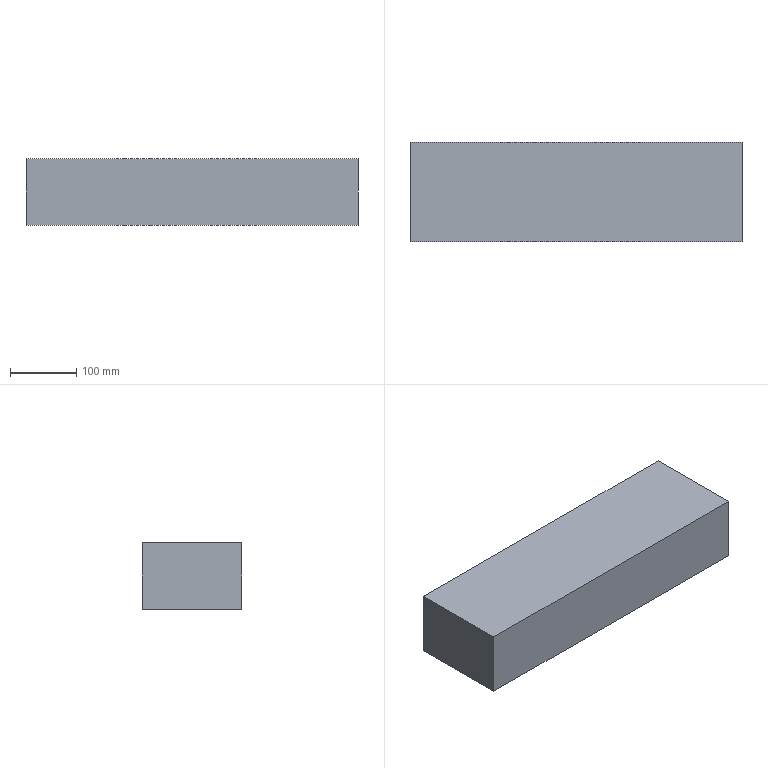Component | SolidWorks | ShadowlessLamp-B-1 | 1 solid | 6 faces | box 500 x 150 x 100 mm | volume 7500000 mm3 | plane 6
build123d program:
from build123d import *

# Parameters (mm, degrees)
SKETCH1_W           = 500
SKETCH1_H           = 100
BOSS_EXTRUDE1_DEPTH = 150


with BuildPart() as part:
    # Sketch1 → Boss-Extrude1 (new body)
    with BuildSketch(Plane.XY):
        Rectangle(SKETCH1_W, SKETCH1_H)
    extrude(amount=BOSS_EXTRUDE1_DEPTH)


solid = part.part

# Placed as in the assembly
solid = solid.moved(Location((-443.006, -571.913, -2307.928), (90, 0, 0)))
STEP:
#1=COLOUR_RGB('',0.7922,0.8196,0.9333);
#2=FILL_AREA_STYLE_COLOUR('',#1);
#3=FILL_AREA_STYLE('',(#2));
#4=SURFACE_STYLE_FILL_AREA(#3);
#5=SURFACE_SIDE_STYLE('',(#4));
#6=SURFACE_STYLE_USAGE(.BOTH.,#5);
#7=PRESENTATION_STYLE_ASSIGNMENT((#6));
#8=CARTESIAN_POINT('',(-7.599,-22.516,-92.832));
#9=VERTEX_POINT('',#8);
#10=CARTESIAN_POINT('',(-7.599,-22.516,-88.895));
#11=VERTEX_POINT('',#10);
#12=CARTESIAN_POINT('',(-7.599,-22.516,-88.895));
#13=DIRECTION('',(0.,-0.,1.));
#14=VECTOR('',#13,39.37);
#15=LINE('',#12,#14);
#16=EDGE_CURVE('',#9,#11,#15,.T.);
#17=ORIENTED_EDGE('',*,*,#16,.T.);
#18=CARTESIAN_POINT('',(-7.599,-28.422,-88.895));
#19=VERTEX_POINT('',#18);
#20=CARTESIAN_POINT('',(-7.599,-28.422,-88.895));
#21=DIRECTION('',(0.,1.,0.));
#22=VECTOR('',#21,39.37);
#23=LINE('',#20,#22);
#24=EDGE_CURVE('',#19,#11,#23,.T.);
#25=ORIENTED_EDGE('',*,*,#24,.F.);
#26=CARTESIAN_POINT('',(-7.599,-28.422,-92.832));
#27=VERTEX_POINT('',#26);
#28=CARTESIAN_POINT('',(-7.599,-28.422,-88.895));
#29=DIRECTION('',(0.,-0.,1.));
#30=VECTOR('',#29,39.37);
#31=LINE('',#28,#30);
#32=EDGE_CURVE('',#27,#19,#31,.T.);
#33=ORIENTED_EDGE('',*,*,#32,.F.);
#34=CARTESIAN_POINT('',(-7.599,-28.422,-92.832));
#35=DIRECTION('',(0.,1.,0.));
#36=VECTOR('',#35,39.37);
#37=LINE('',#34,#36);
#38=EDGE_CURVE('',#27,#9,#37,.T.);
#39=ORIENTED_EDGE('',*,*,#38,.T.);
#40=EDGE_LOOP('',(#17,#25,#33,#39));
#41=FACE_OUTER_BOUND('',#40,.T.);
#42=CARTESIAN_POINT('',(-7.599,-28.422,-88.895));
#43=DIRECTION('',(-1.,0.,0.));
#44=DIRECTION('',(-0.,-1.,-0.));
#45=AXIS2_PLACEMENT_3D('',#42,#43,#44);
#46=PLANE('',#45);
#47=ADVANCED_FACE('',(#41),#46,.F.);
#48=CARTESIAN_POINT('',(-27.284,-22.516,-88.895));
#49=VERTEX_POINT('',#48);
#50=CARTESIAN_POINT('',(-27.284,-22.516,-88.895));
#51=DIRECTION('',(-1.,0.,0.));
#52=VECTOR('',#51,39.37);
#53=LINE('',#50,#52);
#54=EDGE_CURVE('',#11,#49,#53,.T.);
#55=ORIENTED_EDGE('',*,*,#54,.T.);
#56=CARTESIAN_POINT('',(-27.284,-28.422,-88.895));
#57=VERTEX_POINT('',#56);
#58=CARTESIAN_POINT('',(-27.284,-28.422,-88.895));
#59=DIRECTION('',(0.,1.,0.));
#60=VECTOR('',#59,39.37);
#61=LINE('',#58,#60);
#62=EDGE_CURVE('',#57,#49,#61,.T.);
#63=ORIENTED_EDGE('',*,*,#62,.F.);
#64=CARTESIAN_POINT('',(-27.284,-28.422,-88.895));
#65=DIRECTION('',(-1.,0.,0.));
#66=VECTOR('',#65,39.37);
#67=LINE('',#64,#66);
#68=EDGE_CURVE('',#19,#57,#67,.T.);
#69=ORIENTED_EDGE('',*,*,#68,.F.);
#70=ORIENTED_EDGE('',*,*,#24,.T.);
#71=EDGE_LOOP('',(#55,#63,#69,#70));
#72=FACE_OUTER_BOUND('',#71,.T.);
#73=CARTESIAN_POINT('',(-27.284,-28.422,-88.895));
#74=DIRECTION('',(-0.,0.,-1.));
#75=DIRECTION('',(0.,1.,0.));
#76=AXIS2_PLACEMENT_3D('',#73,#74,#75);
#77=PLANE('',#76);
#78=ADVANCED_FACE('',(#72),#77,.F.);
#79=CARTESIAN_POINT('',(-27.284,-22.516,-92.832));
#80=VERTEX_POINT('',#79);
#81=CARTESIAN_POINT('',(-27.284,-22.516,-88.895));
#82=DIRECTION('',(-0.,0.,-1.));
#83=VECTOR('',#82,39.37);
#84=LINE('',#81,#83);
#85=EDGE_CURVE('',#49,#80,#84,.T.);
#86=ORIENTED_EDGE('',*,*,#85,.T.);
#87=CARTESIAN_POINT('',(-27.284,-28.422,-92.832));
#88=VERTEX_POINT('',#87);
#89=CARTESIAN_POINT('',(-27.284,-28.422,-92.832));
#90=DIRECTION('',(0.,1.,0.));
#91=VECTOR('',#90,39.37);
#92=LINE('',#89,#91);
#93=EDGE_CURVE('',#88,#80,#92,.T.);
#94=ORIENTED_EDGE('',*,*,#93,.F.);
#95=CARTESIAN_POINT('',(-27.284,-28.422,-88.895));
#96=DIRECTION('',(-0.,0.,-1.));
#97=VECTOR('',#96,39.37);
#98=LINE('',#95,#97);
#99=EDGE_CURVE('',#57,#88,#98,.T.);
#100=ORIENTED_EDGE('',*,*,#99,.F.);
#101=ORIENTED_EDGE('',*,*,#62,.T.);
#102=EDGE_LOOP('',(#86,#94,#100,#101));
#103=FACE_OUTER_BOUND('',#102,.T.);
#104=CARTESIAN_POINT('',(-27.284,-28.422,-88.895));
#105=DIRECTION('',(1.,-0.,-0.));
#106=DIRECTION('',(0.,1.,0.));
#107=AXIS2_PLACEMENT_3D('',#104,#105,#106);
#108=PLANE('',#107);
#109=ADVANCED_FACE('',(#103),#108,.F.);
#110=CARTESIAN_POINT('',(-27.284,-22.516,-92.832));
#111=DIRECTION('',(1.,-0.,-0.));
#112=VECTOR('',#111,39.37);
#113=LINE('',#110,#112);
#114=EDGE_CURVE('',#80,#9,#113,.T.);
#115=ORIENTED_EDGE('',*,*,#114,.T.);
#116=ORIENTED_EDGE('',*,*,#38,.F.);
#117=CARTESIAN_POINT('',(-27.284,-28.422,-92.832));
#118=DIRECTION('',(1.,-0.,-0.));
#119=VECTOR('',#118,39.37);
#120=LINE('',#117,#119);
#121=EDGE_CURVE('',#88,#27,#120,.T.);
#122=ORIENTED_EDGE('',*,*,#121,.F.);
#123=ORIENTED_EDGE('',*,*,#93,.T.);
#124=EDGE_LOOP('',(#115,#116,#122,#123));
#125=FACE_OUTER_BOUND('',#124,.T.);
#126=CARTESIAN_POINT('',(-27.284,-28.422,-92.832));
#127=DIRECTION('',(0.,-0.,1.));
#128=DIRECTION('',(-0.,-1.,-0.));
#129=AXIS2_PLACEMENT_3D('',#126,#127,#128);
#130=PLANE('',#129);
#131=ADVANCED_FACE('',(#125),#130,.F.);
#132=ORIENTED_EDGE('',*,*,#32,.T.);
#133=ORIENTED_EDGE('',*,*,#68,.T.);
#134=ORIENTED_EDGE('',*,*,#99,.T.);
#135=ORIENTED_EDGE('',*,*,#121,.T.);
#136=EDGE_LOOP('',(#132,#133,#134,#135));
#137=FACE_OUTER_BOUND('',#136,.T.);
#138=CARTESIAN_POINT('',(-17.441,-28.422,-90.863));
#139=DIRECTION('',(-0.,-1.,-0.));
#140=DIRECTION('',(1.,-0.,-0.));
#141=AXIS2_PLACEMENT_3D('',#138,#139,#140);
#142=PLANE('',#141);
#143=ADVANCED_FACE('',(#137),#142,.T.);
#144=ORIENTED_EDGE('',*,*,#16,.F.);
#145=ORIENTED_EDGE('',*,*,#114,.F.);
#146=ORIENTED_EDGE('',*,*,#85,.F.);
#147=ORIENTED_EDGE('',*,*,#54,.F.);
#148=EDGE_LOOP('',(#144,#145,#146,#147));
#149=FACE_OUTER_BOUND('',#148,.T.);
#150=CARTESIAN_POINT('',(-17.441,-22.516,-90.863));
#151=DIRECTION('',(-0.,-1.,-0.));
#152=DIRECTION('',(1.,-0.,-0.));
#153=AXIS2_PLACEMENT_3D('',#150,#151,#152);
#154=PLANE('',#153);
#155=ADVANCED_FACE('',(#149),#154,.F.);
#156=CLOSED_SHELL('',(#47,#78,#109,#131,#143,#155));
#157=MANIFOLD_SOLID_BREP('',#156);
#158=STYLED_ITEM('',(#7),#157);
#159=PRESENTATION_LAYER_ASSIGNMENT('','',(#158));
#160=(LENGTH_UNIT()NAMED_UNIT(*)SI_UNIT($,.METRE.));
#161=LENGTH_MEASURE_WITH_UNIT(LENGTH_MEASURE(0.0254),#160);
#162=DIMENSIONAL_EXPONENTS(1.,0.,0.,0.,0.,0.,0.);
#163=(CONVERSION_BASED_UNIT('',#161)LENGTH_UNIT()NAMED_UNIT(#162));
#164=UNCERTAINTY_MEASURE_WITH_UNIT(LENGTH_MEASURE(0.00001),#163,'','');
#165=(NAMED_UNIT(*)PLANE_ANGLE_UNIT()SI_UNIT($,.RADIAN.));
#166=(NAMED_UNIT(*)SI_UNIT($,.STERADIAN.)SOLID_ANGLE_UNIT());
#167=(GEOMETRIC_REPRESENTATION_CONTEXT(3)GLOBAL_UNCERTAINTY_ASSIGNED_CONTEXT((#164))GLOBAL_UNIT_ASSIGNED_CONTEXT((#163,#165,#166))REPRESENTATION_CONTEXT('',''));
#168=MECHANICAL_DESIGN_GEOMETRIC_PRESENTATION_REPRESENTATION('',(#158),#167);
#169=CARTESIAN_POINT('',(0.,0.,0.));
#170=DIRECTION('',(0.,0.,1.));
#171=DIRECTION('',(1.,0.,0.));
#172=AXIS2_PLACEMENT_3D('',#169,#170,#171);
#173=(LENGTH_UNIT()NAMED_UNIT(*)SI_UNIT($,.METRE.));
#174=LENGTH_MEASURE_WITH_UNIT(LENGTH_MEASURE(0.0254),#173);
#175=DIMENSIONAL_EXPONENTS(1.,0.,0.,0.,0.,0.,0.);
#176=(CONVERSION_BASED_UNIT('',#174)LENGTH_UNIT()NAMED_UNIT(#175));
#177=UNCERTAINTY_MEASURE_WITH_UNIT(LENGTH_MEASURE(0.00001),#176,'','');
#178=(NAMED_UNIT(*)PLANE_ANGLE_UNIT()SI_UNIT($,.RADIAN.));
#179=(NAMED_UNIT(*)SI_UNIT($,.STERADIAN.)SOLID_ANGLE_UNIT());
#180=(GEOMETRIC_REPRESENTATION_CONTEXT(3)GLOBAL_UNCERTAINTY_ASSIGNED_CONTEXT((#177))GLOBAL_UNIT_ASSIGNED_CONTEXT((#176,#178,#179))REPRESENTATION_CONTEXT('',''));
#181=ADVANCED_BREP_SHAPE_REPRESENTATION('',(#157,#172),#180);